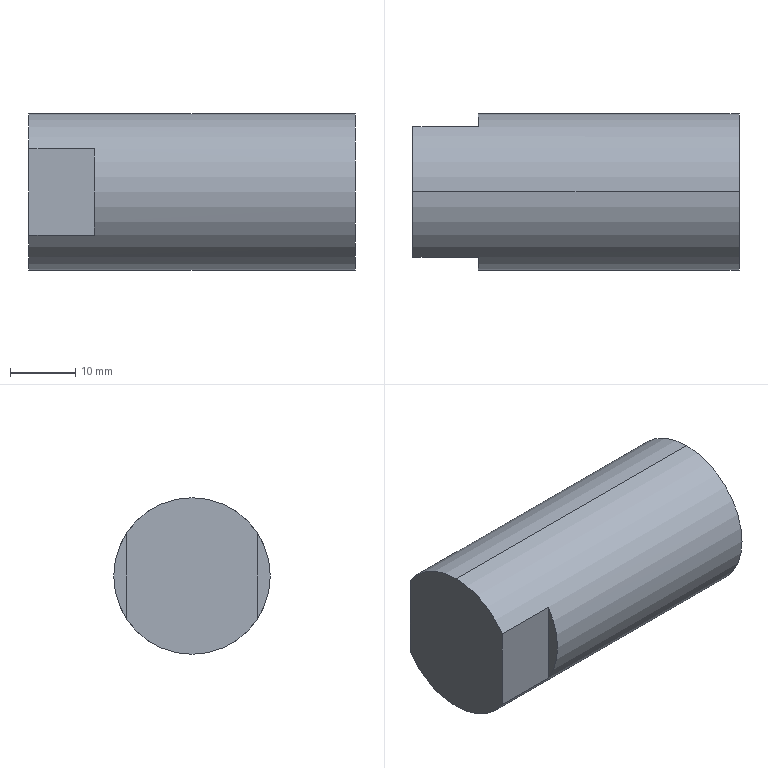Component | SolidWorks | ClampingAssembly-2_24OpticalAxis-1 | 1 solid | 12 faces | box 50 x 24 x 24 mm | volume 20821 mm3 | plane 6 | cylinder 4 | cone 2 | commonest cylinder face diameters 8.5 x2 24 x2 | material 45
build123d program:
from build123d import *

# Parameters (mm, degrees)
SKETCH1_R              = 12
BOSS_EXTRUDE1_DEPTH    = 50
M10_TAPPED_HOLE1_D     = 8.5
M10_TAPPED_HOLE1_DEPTH = 24.5
M10_TAPPED_HOLE1_TIP   = 2.554
SKETCH3_OUTSIDE_W      = 38.086
SKETCH3_OUTSIDE_H      = 38.086
SKETCH3_OUTSIDE_W_2    = 29.211
SKETCH3_OUTSIDE_H_2    = 20
CUT_EXTRUDE1_DEPTH     = 10


with BuildPart() as part:
    # Sketch1 → Boss-Extrude1 (new body)
    with BuildSketch(Plane.XY):
        Circle(SKETCH1_R)
    extrude(amount=BOSS_EXTRUDE1_DEPTH)

    # M10 Tapped Hole1
    with Locations(Plane.XY.offset(50)):
        with Locations((0, 0)):
            Hole(M10_TAPPED_HOLE1_D / 2, depth=M10_TAPPED_HOLE1_DEPTH)
            with Locations((0, 0, -(M10_TAPPED_HOLE1_DEPTH + M10_TAPPED_HOLE1_TIP / 2))):  # 118° drill point
                Cone(0, M10_TAPPED_HOLE1_D / 2, M10_TAPPED_HOLE1_TIP, mode=Mode.SUBTRACT)

    # Sketch3 outside → Cut-Extrude1 (cut)
    with BuildSketch(Plane.XY):
        Rectangle(SKETCH3_OUTSIDE_W, SKETCH3_OUTSIDE_H)
        Rectangle(SKETCH3_OUTSIDE_W_2, SKETCH3_OUTSIDE_H_2, mode=Mode.SUBTRACT)
    extrude(amount=CUT_EXTRUDE1_DEPTH, mode=Mode.SUBTRACT)


solid = part.part

# Placed as in the assembly
solid = solid.moved(Location((-184.365, 21.083, -1210.457), (0, 90, 0)))
STEP:
#1=COLOUR_RGB('',0.7922,0.8196,0.9333);
#2=FILL_AREA_STYLE_COLOUR('',#1);
#3=FILL_AREA_STYLE('',(#2));
#4=SURFACE_STYLE_FILL_AREA(#3);
#5=SURFACE_SIDE_STYLE('',(#4));
#6=SURFACE_STYLE_USAGE(.BOTH.,#5);
#7=PRESENTATION_STYLE_ASSIGNMENT((#6));
#8=CARTESIAN_POINT('',(-6.255,0.83,-47.823));
#9=VERTEX_POINT('',#8);
#10=CARTESIAN_POINT('',(-6.255,0.83,-47.488));
#11=VERTEX_POINT('',#10);
#12=CARTESIAN_POINT('',(-6.255,0.83,-47.656));
#13=DIRECTION('',(1.,-0.,0.));
#14=DIRECTION('',(0.,-0.,1.));
#15=AXIS2_PLACEMENT_3D('',#12,#13,#14);
#16=CIRCLE('',#15,0.1673);
#17=EDGE_CURVE('',#9,#11,#16,.T.);
#18=ORIENTED_EDGE('',*,*,#17,.F.);
#19=CARTESIAN_POINT('',(-5.29,0.83,-47.823));
#20=VERTEX_POINT('',#19);
#21=CARTESIAN_POINT('',(-5.29,0.83,-47.823));
#22=DIRECTION('',(1.,-0.,0.));
#23=VECTOR('',#22,39.37);
#24=LINE('',#21,#23);
#25=EDGE_CURVE('',#9,#20,#24,.T.);
#26=ORIENTED_EDGE('',*,*,#25,.T.);
#27=CARTESIAN_POINT('',(-5.29,0.83,-47.488));
#28=VERTEX_POINT('',#27);
#29=CARTESIAN_POINT('',(-5.29,0.83,-47.656));
#30=DIRECTION('',(1.,-0.,0.));
#31=DIRECTION('',(0.,-0.,1.));
#32=AXIS2_PLACEMENT_3D('',#29,#30,#31);
#33=CIRCLE('',#32,0.1673);
#34=EDGE_CURVE('',#20,#28,#33,.T.);
#35=ORIENTED_EDGE('',*,*,#34,.T.);
#36=CARTESIAN_POINT('',(-5.29,0.83,-47.488));
#37=DIRECTION('',(1.,-0.,0.));
#38=VECTOR('',#37,39.37);
#39=LINE('',#36,#38);
#40=EDGE_CURVE('',#11,#28,#39,.T.);
#41=ORIENTED_EDGE('',*,*,#40,.F.);
#42=EDGE_LOOP('',(#18,#26,#35,#41));
#43=FACE_OUTER_BOUND('',#42,.T.);
#44=CARTESIAN_POINT('',(-5.29,0.83,-47.656));
#45=DIRECTION('',(1.,-0.,0.));
#46=DIRECTION('',(0.,-0.,1.));
#47=AXIS2_PLACEMENT_3D('',#44,#45,#46);
#48=CYLINDRICAL_SURFACE('',#47,0.1673);
#49=ADVANCED_FACE('',(#43),#48,.F.);
#50=CARTESIAN_POINT('',(-6.355,0.83,-47.656));
#51=VERTEX_POINT('',#50);
#52=CARTESIAN_POINT('',(-6.255,0.83,-47.488));
#53=DIRECTION('',(0.515,-0.,0.8572));
#54=VECTOR('',#53,39.37);
#55=LINE('',#52,#54);
#56=EDGE_CURVE('',#51,#11,#55,.T.);
#57=ORIENTED_EDGE('',*,*,#56,.F.);
#58=CARTESIAN_POINT('',(-6.255,0.83,-47.823));
#59=DIRECTION('',(0.515,0.,-0.8572));
#60=VECTOR('',#59,39.37);
#61=LINE('',#58,#60);
#62=EDGE_CURVE('',#51,#9,#61,.T.);
#63=ORIENTED_EDGE('',*,*,#62,.T.);
#64=ORIENTED_EDGE('',*,*,#17,.T.);
#65=EDGE_LOOP('',(#57,#63,#64));
#66=FACE_OUTER_BOUND('',#65,.T.);
#67=CARTESIAN_POINT('',(-6.255,0.83,-47.656));
#68=DIRECTION('',(1.,-0.,0.));
#69=DIRECTION('',(0.,-0.,1.));
#70=AXIS2_PLACEMENT_3D('',#67,#68,#69);
#71=CONICAL_SURFACE('',#70,0.1673,1.03);
#72=ADVANCED_FACE('',(#66),#71,.F.);
#73=CARTESIAN_POINT('',(-5.29,0.83,-47.183));
#74=VERTEX_POINT('',#73);
#75=CARTESIAN_POINT('',(-5.29,0.83,-48.128));
#76=VERTEX_POINT('',#75);
#77=CARTESIAN_POINT('',(-5.29,0.83,-47.656));
#78=DIRECTION('',(1.,-0.,0.));
#79=DIRECTION('',(0.,-0.,1.));
#80=AXIS2_PLACEMENT_3D('',#77,#78,#79);
#81=CIRCLE('',#80,0.4724);
#82=EDGE_CURVE('',#74,#76,#81,.T.);
#83=ORIENTED_EDGE('',*,*,#82,.F.);
#84=CARTESIAN_POINT('',(-7.258,0.83,-47.183));
#85=VERTEX_POINT('',#84);
#86=CARTESIAN_POINT('',(-5.29,0.83,-47.183));
#87=DIRECTION('',(-1.,0.,-0.));
#88=VECTOR('',#87,39.37);
#89=LINE('',#86,#88);
#90=EDGE_CURVE('',#74,#85,#89,.T.);
#91=ORIENTED_EDGE('',*,*,#90,.T.);
#92=CARTESIAN_POINT('',(-7.258,0.4363,-47.395));
#93=VERTEX_POINT('',#92);
#94=CARTESIAN_POINT('',(-7.258,0.83,-47.656));
#95=DIRECTION('',(1.,-0.,0.));
#96=DIRECTION('',(0.,-0.,1.));
#97=AXIS2_PLACEMENT_3D('',#94,#95,#96);
#98=CIRCLE('',#97,0.4724);
#99=EDGE_CURVE('',#85,#93,#98,.T.);
#100=ORIENTED_EDGE('',*,*,#99,.T.);
#101=CARTESIAN_POINT('',(-6.865,0.4363,-47.395));
#102=VERTEX_POINT('',#101);
#103=CARTESIAN_POINT('',(-5.29,0.4363,-47.395));
#104=DIRECTION('',(1.,-0.,0.));
#105=VECTOR('',#104,39.37);
#106=LINE('',#103,#105);
#107=EDGE_CURVE('',#93,#102,#106,.T.);
#108=ORIENTED_EDGE('',*,*,#107,.T.);
#109=CARTESIAN_POINT('',(-6.865,0.4363,-47.917));
#110=VERTEX_POINT('',#109);
#111=CARTESIAN_POINT('',(-6.865,0.83,-47.656));
#112=DIRECTION('',(1.,-0.,0.));
#113=DIRECTION('',(0.,-0.,1.));
#114=AXIS2_PLACEMENT_3D('',#111,#112,#113);
#115=CIRCLE('',#114,0.4724);
#116=EDGE_CURVE('',#102,#110,#115,.T.);
#117=ORIENTED_EDGE('',*,*,#116,.T.);
#118=CARTESIAN_POINT('',(-7.258,0.4363,-47.917));
#119=VERTEX_POINT('',#118);
#120=CARTESIAN_POINT('',(-5.29,0.4363,-47.917));
#121=DIRECTION('',(-1.,0.,-0.));
#122=VECTOR('',#121,39.37);
#123=LINE('',#120,#122);
#124=EDGE_CURVE('',#110,#119,#123,.T.);
#125=ORIENTED_EDGE('',*,*,#124,.T.);
#126=CARTESIAN_POINT('',(-7.258,0.83,-48.128));
#127=VERTEX_POINT('',#126);
#128=CARTESIAN_POINT('',(-7.258,0.83,-47.656));
#129=DIRECTION('',(1.,-0.,0.));
#130=DIRECTION('',(0.,-0.,1.));
#131=AXIS2_PLACEMENT_3D('',#128,#129,#130);
#132=CIRCLE('',#131,0.4724);
#133=EDGE_CURVE('',#119,#127,#132,.T.);
#134=ORIENTED_EDGE('',*,*,#133,.T.);
#135=CARTESIAN_POINT('',(-5.29,0.83,-48.128));
#136=DIRECTION('',(-1.,0.,-0.));
#137=VECTOR('',#136,39.37);
#138=LINE('',#135,#137);
#139=EDGE_CURVE('',#76,#127,#138,.T.);
#140=ORIENTED_EDGE('',*,*,#139,.F.);
#141=EDGE_LOOP('',(#83,#91,#100,#108,#117,#125,#134,#140));
#142=FACE_OUTER_BOUND('',#141,.T.);
#143=CARTESIAN_POINT('',(-5.29,0.83,-47.656));
#144=DIRECTION('',(-1.,0.,-0.));
#145=DIRECTION('',(0.,0.,-1.));
#146=AXIS2_PLACEMENT_3D('',#143,#144,#145);
#147=CYLINDRICAL_SURFACE('',#146,0.4724);
#148=ADVANCED_FACE('',(#142),#147,.T.);
#149=ORIENTED_EDGE('',*,*,#90,.F.);
#150=CARTESIAN_POINT('',(-5.29,0.83,-47.656));
#151=DIRECTION('',(1.,-0.,0.));
#152=DIRECTION('',(0.,-0.,1.));
#153=AXIS2_PLACEMENT_3D('',#150,#151,#152);
#154=CIRCLE('',#153,0.4724);
#155=EDGE_CURVE('',#76,#74,#154,.T.);
#156=ORIENTED_EDGE('',*,*,#155,.F.);
#157=ORIENTED_EDGE('',*,*,#139,.T.);
#158=CARTESIAN_POINT('',(-7.258,1.224,-47.917));
#159=VERTEX_POINT('',#158);
#160=CARTESIAN_POINT('',(-7.258,0.83,-47.656));
#161=DIRECTION('',(1.,-0.,0.));
#162=DIRECTION('',(0.,-0.,1.));
#163=AXIS2_PLACEMENT_3D('',#160,#161,#162);
#164=CIRCLE('',#163,0.4724);
#165=EDGE_CURVE('',#127,#159,#164,.T.);
#166=ORIENTED_EDGE('',*,*,#165,.T.);
#167=CARTESIAN_POINT('',(-6.865,1.224,-47.917));
#168=VERTEX_POINT('',#167);
#169=CARTESIAN_POINT('',(-5.29,1.224,-47.917));
#170=DIRECTION('',(1.,-0.,0.));
#171=VECTOR('',#170,39.37);
#172=LINE('',#169,#171);
#173=EDGE_CURVE('',#159,#168,#172,.T.);
#174=ORIENTED_EDGE('',*,*,#173,.T.);
#175=CARTESIAN_POINT('',(-6.865,1.224,-47.395));
#176=VERTEX_POINT('',#175);
#177=CARTESIAN_POINT('',(-6.865,0.83,-47.656));
#178=DIRECTION('',(1.,-0.,0.));
#179=DIRECTION('',(0.,-0.,1.));
#180=AXIS2_PLACEMENT_3D('',#177,#178,#179);
#181=CIRCLE('',#180,0.4724);
#182=EDGE_CURVE('',#168,#176,#181,.T.);
#183=ORIENTED_EDGE('',*,*,#182,.T.);
#184=CARTESIAN_POINT('',(-7.258,1.224,-47.395));
#185=VERTEX_POINT('',#184);
#186=CARTESIAN_POINT('',(-5.29,1.224,-47.395));
#187=DIRECTION('',(-1.,0.,-0.));
#188=VECTOR('',#187,39.37);
#189=LINE('',#186,#188);
#190=EDGE_CURVE('',#176,#185,#189,.T.);
#191=ORIENTED_EDGE('',*,*,#190,.T.);
#192=CARTESIAN_POINT('',(-7.258,0.83,-47.656));
#193=DIRECTION('',(1.,-0.,0.));
#194=DIRECTION('',(0.,-0.,1.));
#195=AXIS2_PLACEMENT_3D('',#192,#193,#194);
#196=CIRCLE('',#195,0.4724);
#197=EDGE_CURVE('',#185,#85,#196,.T.);
#198=ORIENTED_EDGE('',*,*,#197,.T.);
#199=EDGE_LOOP('',(#149,#156,#157,#166,#174,#183,#191,#198));
#200=FACE_OUTER_BOUND('',#199,.T.);
#201=CARTESIAN_POINT('',(-5.29,0.83,-47.656));
#202=DIRECTION('',(-1.,0.,-0.));
#203=DIRECTION('',(0.,0.,-1.));
#204=AXIS2_PLACEMENT_3D('',#201,#202,#203);
#205=CYLINDRICAL_SURFACE('',#204,0.4724);
#206=ADVANCED_FACE('',(#200),#205,.T.);
#207=CARTESIAN_POINT('',(-5.29,0.83,-47.656));
#208=DIRECTION('',(1.,-0.,0.));
#209=DIRECTION('',(0.,-0.,1.));
#210=AXIS2_PLACEMENT_3D('',#207,#208,#209);
#211=CIRCLE('',#210,0.1673);
#212=EDGE_CURVE('',#28,#20,#211,.T.);
#213=ORIENTED_EDGE('',*,*,#212,.F.);
#214=ORIENTED_EDGE('',*,*,#34,.F.);
#215=EDGE_LOOP('',(#213,#214));
#216=FACE_BOUND('',#215,.T.);
#217=ORIENTED_EDGE('',*,*,#155,.T.);
#218=ORIENTED_EDGE('',*,*,#82,.T.);
#219=EDGE_LOOP('',(#217,#218));
#220=FACE_OUTER_BOUND('',#219,.T.);
#221=CARTESIAN_POINT('',(-5.29,0.83,-47.656));
#222=DIRECTION('',(1.,-0.,0.));
#223=DIRECTION('',(-0.,-0.,1.));
#224=AXIS2_PLACEMENT_3D('',#221,#222,#223);
#225=PLANE('',#224);
#226=ADVANCED_FACE('',(#216,#220),#225,.T.);
#227=ORIENTED_EDGE('',*,*,#133,.F.);
#228=CARTESIAN_POINT('',(-7.258,0.4363,-47.656));
#229=DIRECTION('',(-0.,-0.,1.));
#230=VECTOR('',#229,39.37);
#231=LINE('',#228,#230);
#232=EDGE_CURVE('',#119,#93,#231,.T.);
#233=ORIENTED_EDGE('',*,*,#232,.T.);
#234=ORIENTED_EDGE('',*,*,#99,.F.);
#235=ORIENTED_EDGE('',*,*,#197,.F.);
#236=CARTESIAN_POINT('',(-7.258,1.224,-47.656));
#237=DIRECTION('',(0.,0.,-1.));
#238=VECTOR('',#237,39.37);
#239=LINE('',#236,#238);
#240=EDGE_CURVE('',#185,#159,#239,.T.);
#241=ORIENTED_EDGE('',*,*,#240,.T.);
#242=ORIENTED_EDGE('',*,*,#165,.F.);
#243=EDGE_LOOP('',(#227,#233,#234,#235,#241,#242));
#244=FACE_OUTER_BOUND('',#243,.T.);
#245=CARTESIAN_POINT('',(-7.258,0.83,-47.656));
#246=DIRECTION('',(1.,-0.,0.));
#247=DIRECTION('',(-0.,-0.,1.));
#248=AXIS2_PLACEMENT_3D('',#245,#246,#247);
#249=PLANE('',#248);
#250=ADVANCED_FACE('',(#244),#249,.F.);
#251=ORIENTED_EDGE('',*,*,#62,.F.);
#252=ORIENTED_EDGE('',*,*,#56,.T.);
#253=CARTESIAN_POINT('',(-6.255,0.83,-47.656));
#254=DIRECTION('',(1.,-0.,0.));
#255=DIRECTION('',(0.,-0.,1.));
#256=AXIS2_PLACEMENT_3D('',#253,#254,#255);
#257=CIRCLE('',#256,0.1673);
#258=EDGE_CURVE('',#11,#9,#257,.T.);
#259=ORIENTED_EDGE('',*,*,#258,.T.);
#260=EDGE_LOOP('',(#251,#252,#259));
#261=FACE_OUTER_BOUND('',#260,.T.);
#262=CARTESIAN_POINT('',(-6.255,0.83,-47.656));
#263=DIRECTION('',(1.,-0.,0.));
#264=DIRECTION('',(0.,-0.,1.));
#265=AXIS2_PLACEMENT_3D('',#262,#263,#264);
#266=CONICAL_SURFACE('',#265,0.1673,1.03);
#267=ADVANCED_FACE('',(#261),#266,.F.);
#268=ORIENTED_EDGE('',*,*,#25,.F.);
#269=ORIENTED_EDGE('',*,*,#258,.F.);
#270=ORIENTED_EDGE('',*,*,#40,.T.);
#271=ORIENTED_EDGE('',*,*,#212,.T.);
#272=EDGE_LOOP('',(#268,#269,#270,#271));
#273=FACE_OUTER_BOUND('',#272,.T.);
#274=CARTESIAN_POINT('',(-5.29,0.83,-47.656));
#275=DIRECTION('',(1.,-0.,0.));
#276=DIRECTION('',(0.,-0.,1.));
#277=AXIS2_PLACEMENT_3D('',#274,#275,#276);
#278=CYLINDRICAL_SURFACE('',#277,0.1673);
#279=ADVANCED_FACE('',(#273),#278,.F.);
#280=CARTESIAN_POINT('',(-6.865,1.224,-48.231));
#281=DIRECTION('',(-0.,-0.,1.));
#282=VECTOR('',#281,39.37);
#283=LINE('',#280,#282);
#284=EDGE_CURVE('',#168,#176,#283,.T.);
#285=ORIENTED_EDGE('',*,*,#284,.F.);
#286=ORIENTED_EDGE('',*,*,#173,.F.);
#287=ORIENTED_EDGE('',*,*,#240,.F.);
#288=ORIENTED_EDGE('',*,*,#190,.F.);
#289=EDGE_LOOP('',(#285,#286,#287,#288));
#290=FACE_OUTER_BOUND('',#289,.T.);
#291=CARTESIAN_POINT('',(-6.865,1.224,-48.231));
#292=DIRECTION('',(-0.,-1.,-0.));
#293=DIRECTION('',(1.,-0.,0.));
#294=AXIS2_PLACEMENT_3D('',#291,#292,#293);
#295=PLANE('',#294);
#296=ADVANCED_FACE('',(#290),#295,.F.);
#297=ORIENTED_EDGE('',*,*,#284,.T.);
#298=ORIENTED_EDGE('',*,*,#182,.F.);
#299=EDGE_LOOP('',(#297,#298));
#300=FACE_OUTER_BOUND('',#299,.T.);
#301=CARTESIAN_POINT('',(-6.865,0.83,-47.656));
#302=DIRECTION('',(1.,-0.,0.));
#303=DIRECTION('',(-0.,-0.,1.));
#304=AXIS2_PLACEMENT_3D('',#301,#302,#303);
#305=PLANE('',#304);
#306=ADVANCED_FACE('',(#300),#305,.F.);
#307=CARTESIAN_POINT('',(-6.865,0.4363,-48.231));
#308=DIRECTION('',(0.,0.,-1.));
#309=VECTOR('',#308,39.37);
#310=LINE('',#307,#309);
#311=EDGE_CURVE('',#102,#110,#310,.T.);
#312=ORIENTED_EDGE('',*,*,#311,.T.);
#313=ORIENTED_EDGE('',*,*,#116,.F.);
#314=EDGE_LOOP('',(#312,#313));
#315=FACE_OUTER_BOUND('',#314,.T.);
#316=CARTESIAN_POINT('',(-6.865,0.83,-47.656));
#317=DIRECTION('',(1.,-0.,0.));
#318=DIRECTION('',(-0.,-0.,1.));
#319=AXIS2_PLACEMENT_3D('',#316,#317,#318);
#320=PLANE('',#319);
#321=ADVANCED_FACE('',(#315),#320,.F.);
#322=ORIENTED_EDGE('',*,*,#311,.F.);
#323=ORIENTED_EDGE('',*,*,#107,.F.);
#324=ORIENTED_EDGE('',*,*,#232,.F.);
#325=ORIENTED_EDGE('',*,*,#124,.F.);
#326=EDGE_LOOP('',(#322,#323,#324,#325));
#327=FACE_OUTER_BOUND('',#326,.T.);
#328=CARTESIAN_POINT('',(-6.865,0.4363,-48.231));
#329=DIRECTION('',(0.,1.,0.));
#330=DIRECTION('',(-1.,0.,-0.));
#331=AXIS2_PLACEMENT_3D('',#328,#329,#330);
#332=PLANE('',#331);
#333=ADVANCED_FACE('',(#327),#332,.F.);
#334=CLOSED_SHELL('',(#49,#72,#148,#206,#226,#250,#267,#279,#296,#306,#321,#333));
#335=MANIFOLD_SOLID_BREP('',#334);
#336=STYLED_ITEM('',(#7),#335);
#337=PRESENTATION_LAYER_ASSIGNMENT('','',(#336));
#338=(LENGTH_UNIT()NAMED_UNIT(*)SI_UNIT($,.METRE.));
#339=LENGTH_MEASURE_WITH_UNIT(LENGTH_MEASURE(0.0254),#338);
#340=DIMENSIONAL_EXPONENTS(1.,0.,0.,0.,0.,0.,0.);
#341=(CONVERSION_BASED_UNIT('',#339)LENGTH_UNIT()NAMED_UNIT(#340));
#342=UNCERTAINTY_MEASURE_WITH_UNIT(LENGTH_MEASURE(0.00001),#341,'','');
#343=(NAMED_UNIT(*)PLANE_ANGLE_UNIT()SI_UNIT($,.RADIAN.));
#344=(NAMED_UNIT(*)SI_UNIT($,.STERADIAN.)SOLID_ANGLE_UNIT());
#345=(GEOMETRIC_REPRESENTATION_CONTEXT(3)GLOBAL_UNCERTAINTY_ASSIGNED_CONTEXT((#342))GLOBAL_UNIT_ASSIGNED_CONTEXT((#341,#343,#344))REPRESENTATION_CONTEXT('',''));
#346=MECHANICAL_DESIGN_GEOMETRIC_PRESENTATION_REPRESENTATION('',(#336),#345);
#347=CARTESIAN_POINT('',(0.,0.,0.));
#348=DIRECTION('',(0.,0.,1.));
#349=DIRECTION('',(1.,0.,0.));
#350=AXIS2_PLACEMENT_3D('',#347,#348,#349);
#351=(LENGTH_UNIT()NAMED_UNIT(*)SI_UNIT($,.METRE.));
#352=LENGTH_MEASURE_WITH_UNIT(LENGTH_MEASURE(0.0254),#351);
#353=DIMENSIONAL_EXPONENTS(1.,0.,0.,0.,0.,0.,0.);
#354=(CONVERSION_BASED_UNIT('',#352)LENGTH_UNIT()NAMED_UNIT(#353));
#355=UNCERTAINTY_MEASURE_WITH_UNIT(LENGTH_MEASURE(0.00001),#354,'','');
#356=(NAMED_UNIT(*)PLANE_ANGLE_UNIT()SI_UNIT($,.RADIAN.));
#357=(NAMED_UNIT(*)SI_UNIT($,.STERADIAN.)SOLID_ANGLE_UNIT());
#358=(GEOMETRIC_REPRESENTATION_CONTEXT(3)GLOBAL_UNCERTAINTY_ASSIGNED_CONTEXT((#355))GLOBAL_UNIT_ASSIGNED_CONTEXT((#354,#356,#357))REPRESENTATION_CONTEXT('',''));
#359=ADVANCED_BREP_SHAPE_REPRESENTATION('',(#335,#350),#358);